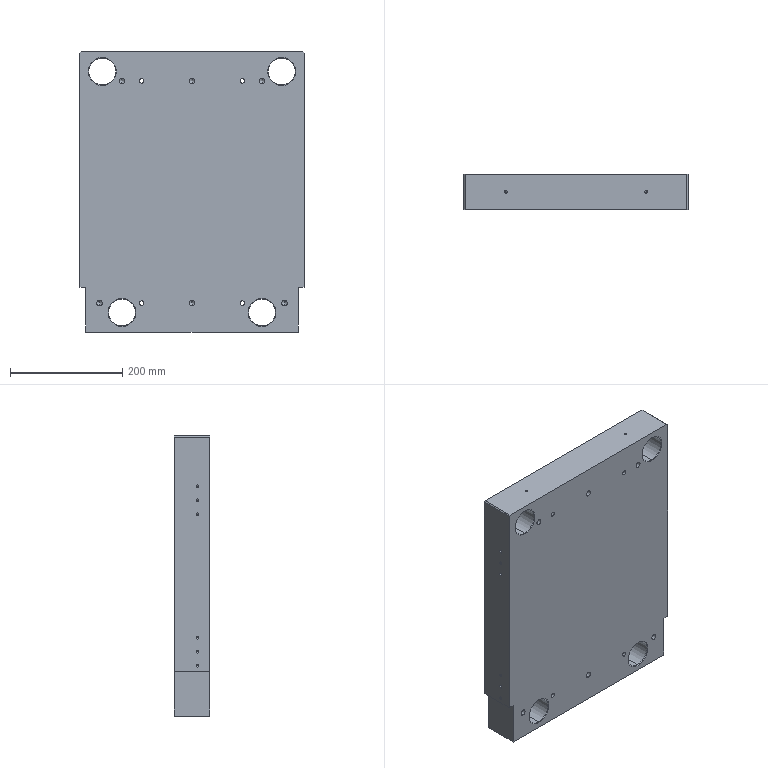Component | SolidWorks | NewDieSet-1_UpperDieSetAssembly-1_KF525R2-MJ-A001-1 | 1 solid | 136 faces | box 400 x 63 x 500 mm | volume 12000457 mm3 | cylinder 64 | cone 60 | plane 12 | commonest cylinder face diameters 5 x32 10.2 x12 8 x8 48 x8 14 x4 | material 55
build123d program:
from build123d import *

# Parameters (mm, degrees)
SKETCH1_W                   = 400
SKETCH1_H                   = 500
BOSS_EXTRUDE1_DEPTH         = 63
SKETCH3_R                   = 24
CUT_EXTRUDE2_DEPTH          = 644.404
CHAMFER1_SIZE               = 1
M6_TAPPED_HOLE1_AT_2_COUNT  = 2
M6_TAPPED_HOLE1_AT_2_PITCH  = 50
M6_TAPPED_HOLE1_AT_3_COUNT  = 2
M6_TAPPED_HOLE1_AT_3_PITCH  = 25
M16_TAPPED_HOLE1_D          = 14
M16_TAPPED_HOLE1_DEPTH      = 30
M16_TAPPED_HOLE1_TIP        = 4.206
M12_TAPPED_HOLE2_AT_2_COUNT = 2
M12_TAPPED_HOLE2_AT_2_PITCH = 165
M12_TAPPED_HOLE2_AT_3_COUNT = 2
M12_TAPPED_HOLE2_AT_3_PITCH = 330
SKETCH45_R                  = 4
CUT_EXTRUDE15_DEPTH         = 644.404
CHAMFER3_SIZE               = 2
SKETCH50_W                  = 10
SKETCH50_H                  = 80
CUT_EXTRUDE17_DEPTH         = 644.404
M6_TAPPED_HOLE3_AT_2_COUNT  = 2
M6_TAPPED_HOLE3_AT_2_PITCH  = 250
M12_TAPPED_HOLE3_D          = 10.2
M12_TAPPED_HOLE3_DEPTH      = 29.25
M12_TAPPED_HOLE3_TIP        = 3.064


with BuildPart() as part:
    # Sketch1 → Boss-Extrude1 (new body)
    with BuildSketch(Plane(origin=(0, 0, 0), x_dir=(1, 0, 0), z_dir=(0, 1, 0))):
        with Locations((200, 250)):
            Rectangle(SKETCH1_W, SKETCH1_H)
    extrude(amount=BOSS_EXTRUDE1_DEPTH)

    # Sketch3 → Cut-Extrude2 (cut, through all)
    with BuildSketch(Plane(origin=(0, 63, 0), x_dir=(1, 0, 0), z_dir=(0, 1, 0))):
        with Locations(Location((75, 465, 0), (0, 0, 270))):
            Circle(SKETCH3_R)
        with Locations(Location((40, 35, 0), (0, 0, 270))):
            Circle(SKETCH3_R)
        with Locations(Location((360, 35, 0), (0, 0, 90))):
            Circle(SKETCH3_R)
        with Locations(Location((325, 465, 0), (0, 0, 90))):
            Circle(SKETCH3_R)
    extrude(amount=-CUT_EXTRUDE2_DEPTH, mode=Mode.SUBTRACT)

    # Chamfer1
    chamfer1_edges = [part.edges().sort_by_distance(p)[0] for p in [
        (75, 0, -489),
        (75, 63, -489),
        (40, 0, -59),
        (40, 63, -59),
        (360, 0, -11),
        (360, 63, -11),
        (325, 0, -441),
        (325, 63, -441),
    ]]
    chamfer(chamfer1_edges, length=CHAMFER1_SIZE)

    # Sketch39 → M6 Tapped Hole1 (revolve, cut)
    with BuildSketch(Plane(origin=(400, 21.5, -140), x_dir=(0, 0, -1), z_dir=(0, 1, 0))):
        Polygon((0, 0), (0, 16.502), (2.5, 15), (2.5, 0), align=None)
    m6_tapped_hole1 = revolve(axis=Axis((406.35, 21.5, -140), (-1, 0, 0)), mode=Mode.SUBTRACT)

    # M6 Tapped Hole1 at 2: M6 Tapped Hole1 ×2
    with Locations(*[(0, 0, i * M6_TAPPED_HOLE1_AT_2_PITCH) for i in range(1, M6_TAPPED_HOLE1_AT_2_COUNT)]):
        add(m6_tapped_hole1, mode=Mode.SUBTRACT)

    # M6 Tapped Hole1 at 3: M6 Tapped Hole1 ×2
    with Locations(*[(0, 0, i * M6_TAPPED_HOLE1_AT_3_PITCH) for i in range(1, M6_TAPPED_HOLE1_AT_3_COUNT)]):
        add(m6_tapped_hole1, mode=Mode.SUBTRACT)

    # Mirror5: M6 Tapped Hole1 across plane
    add(m6_tapped_hole1.mirror(Plane.XY.offset(-250)), mode=Mode.SUBTRACT)

    # Mirror5 copy 1 sketch → Mirror5 copy 1 (revolve, cut)
    with BuildSketch(Plane(origin=(400, 21.5, -410), x_dir=(0, 0, 1), z_dir=(0, 1, 0))):
        Polygon((0, 0), (0, -16.502), (2.5, -15), (2.5, 0), align=None)
    revolve(axis=Axis((406.35, 21.5, -410), (1, 0, 0)), mode=Mode.SUBTRACT)

    # Mirror5 copy 2 sketch → Mirror5 copy 2 (revolve, cut)
    with BuildSketch(Plane(origin=(400, 21.5, -385), x_dir=(0, 0, 1), z_dir=(0, 1, 0))):
        Polygon((0, 0), (0, -16.502), (2.5, -15), (2.5, 0), align=None)
    revolve(axis=Axis((406.35, 21.5, -385), (1, 0, 0)), mode=Mode.SUBTRACT)

    # Mirror6: M6 Tapped Hole1 across plane
    add(m6_tapped_hole1.mirror(Plane.ZY.offset(-200)), mode=Mode.SUBTRACT)

    # Mirror6 copy 1 sketch → Mirror6 copy 1 (revolve, cut)
    with BuildSketch(Plane(origin=(0, 21.5, -90), x_dir=(0, 0, -1), z_dir=(0, 1, 0))):
        Polygon((0, 0), (0, -16.502), (2.5, -15), (2.5, 0), align=None)
    revolve(axis=Axis((-6.35, 21.5, -90), (-1, 0, 0)), mode=Mode.SUBTRACT)

    # Mirror6 copy 2 sketch → Mirror6 copy 2 (revolve, cut)
    with BuildSketch(Plane(origin=(0, 21.5, -115), x_dir=(0, 0, -1), z_dir=(0, 1, 0))):
        Polygon((0, 0), (0, -16.502), (2.5, -15), (2.5, 0), align=None)
    revolve(axis=Axis((-6.35, 21.5, -115), (-1, 0, 0)), mode=Mode.SUBTRACT)

    # Mirror6 copy 3 sketch → Mirror6 copy 3 (revolve, cut)
    with BuildSketch(Plane(origin=(0, 21.5, -360), x_dir=(0, 0, 1), z_dir=(0, 1, 0))):
        Polygon((0, 0), (0, 16.502), (2.5, 15), (2.5, 0), align=None)
    revolve(axis=Axis((-6.35, 21.5, -360), (1, 0, 0)), mode=Mode.SUBTRACT)

    # Mirror6 copy 4 sketch → Mirror6 copy 4 (revolve, cut)
    with BuildSketch(Plane(origin=(0, 21.5, -410), x_dir=(0, 0, 1), z_dir=(0, 1, 0))):
        Polygon((0, 0), (0, 16.502), (2.5, 15), (2.5, 0), align=None)
    revolve(axis=Axis((-6.35, 21.5, -410), (1, 0, 0)), mode=Mode.SUBTRACT)

    # Mirror6 copy 5 sketch → Mirror6 copy 5 (revolve, cut)
    with BuildSketch(Plane(origin=(0, 21.5, -385), x_dir=(0, 0, 1), z_dir=(0, 1, 0))):
        Polygon((0, 0), (0, 16.502), (2.5, 15), (2.5, 0), align=None)
    revolve(axis=Axis((-6.35, 21.5, -385), (1, 0, 0)), mode=Mode.SUBTRACT)

    # M16 Tapped Hole1
    with Locations(Plane(origin=(0, 63, 0), x_dir=(1, 0, 0), z_dir=(0, 1, 0))):
        with Locations((340, 260), (60, 260)):
            Hole(M16_TAPPED_HOLE1_D / 2, depth=M16_TAPPED_HOLE1_DEPTH)
            with Locations((0, 0, -(M16_TAPPED_HOLE1_DEPTH + M16_TAPPED_HOLE1_TIP / 2))):  # 118° drill point
                Cone(0, M16_TAPPED_HOLE1_D / 2, M16_TAPPED_HOLE1_TIP, mode=Mode.SUBTRACT)

    # Sketch43 → M12 Tapped Hole2 (revolve, cut)
    with BuildSketch(Plane(origin=(365, 0, -51.9), x_dir=(0, 0, -1), z_dir=(1, 0, 0))):
        Polygon((0, 0), (0, 32.314), (5.1, 29.25), (5.1, 0), align=None)
    m12_tapped_hole2 = revolve(axis=Axis((365, -6.35, -51.9), (0, 1, 0)), mode=Mode.SUBTRACT)

    # M12 Tapped Hole2 at 2: M12 Tapped Hole2 ×2
    with Locations(*[(-i * M12_TAPPED_HOLE2_AT_2_PITCH, 0, 0) for i in range(1, M12_TAPPED_HOLE2_AT_2_COUNT)]):
        add(m12_tapped_hole2, mode=Mode.SUBTRACT)

    # M12 Tapped Hole2 at 3: M12 Tapped Hole2 ×2
    with Locations(*[(-i * M12_TAPPED_HOLE2_AT_3_PITCH, 0, 0) for i in range(1, M12_TAPPED_HOLE2_AT_3_COUNT)]):
        add(m12_tapped_hole2, mode=Mode.SUBTRACT)

    # Sketch45 → Cut-Extrude15 (cut, through all)
    with BuildSketch(Plane.XZ):
        with Locations(Location((290, -51.9, 0), (0, 0, 270))):
            Circle(SKETCH45_R)
        with Locations(Location((110, -51.9, 0), (0, 0, 270))):
            Circle(SKETCH45_R)
    cut_extrude15 = extrude(amount=-CUT_EXTRUDE15_DEPTH, mode=Mode.SUBTRACT)

    # Mirror7: M12 Tapped Hole2, Cut-Extrude15 across plane
    add(m12_tapped_hole2.mirror(Plane.XY.offset(-250)), mode=Mode.SUBTRACT)
    add(cut_extrude15.mirror(Plane.XY.offset(-250)), mode=Mode.SUBTRACT)

    # Mirror7 copy 1 sketch → Mirror7 copy 1 (revolve, cut)
    with BuildSketch(Plane(origin=(200, 0, -448.1), x_dir=(0, 0, 1), z_dir=(1, 0, 0))):
        Polygon((0, 0), (0, -32.314), (5.1, -29.25), (5.1, 0), align=None)
    revolve(axis=Axis((200, -6.35, -448.1), (0, -1, 0)), mode=Mode.SUBTRACT)

    # Mirror7 copy 2 sketch → Mirror7 copy 2 (revolve, cut)
    with BuildSketch(Plane(origin=(35, 0, -448.1), x_dir=(0, 0, 1), z_dir=(1, 0, 0))):
        Polygon((0, 0), (0, -32.314), (5.1, -29.25), (5.1, 0), align=None)
    revolve(axis=Axis((35, -6.35, -448.1), (0, -1, 0)), mode=Mode.SUBTRACT)

    # Chamfer3
    chamfer3_edges = [part.edges().sort_by_distance(p)[0] for p in [
        (0, 31.5, -500),
        (400, 31.5, -500),
        (400, 31.5, 0),
        (0, 31.5, 0),
    ]]
    chamfer(chamfer3_edges, length=CHAMFER3_SIZE)

    # Sketch50 → Cut-Extrude17 (cut, through all)
    with BuildSketch(Plane(origin=(0, 63, 0), x_dir=(1, 0, 0), z_dir=(0, 1, 0))):
        with Locations((395, 460)):
            Rectangle(SKETCH50_W, SKETCH50_H)
    cut_extrude17 = extrude(amount=-CUT_EXTRUDE17_DEPTH, mode=Mode.SUBTRACT)

    # Mirror9: Cut-Extrude17 across plane
    add(cut_extrude17.mirror(Plane.ZY.offset(-200)), mode=Mode.SUBTRACT)

    # Sketch51 → M6 Tapped Hole3 (revolve, cut)
    with BuildSketch(Plane(origin=(75, 31.5, -500), x_dir=(0, 1, 0), z_dir=(1, 0, 0))):
        Polygon((0, 0), (0, 16.502), (2.5, 15), (2.5, 0), align=None)
    m6_tapped_hole3 = revolve(axis=Axis((75, 31.5, -506.35), (0, 0, 1)), mode=Mode.SUBTRACT)

    # M6 Tapped Hole3 at 2: M6 Tapped Hole3 ×2
    with Locations(*[(i * M6_TAPPED_HOLE3_AT_2_PITCH, 0, 0) for i in range(1, M6_TAPPED_HOLE3_AT_2_COUNT)]):
        add(m6_tapped_hole3, mode=Mode.SUBTRACT)

    # Mirror10: M6 Tapped Hole3 across plane
    add(m6_tapped_hole3.mirror(Plane.XY.offset(-250)), mode=Mode.SUBTRACT)

    # Mirror10 copy 1 sketch → Mirror10 copy 1 (revolve, cut)
    with BuildSketch(Plane(origin=(325, 31.5, 0), x_dir=(0, 1, 0), z_dir=(1, 0, 0))):
        Polygon((0, 0), (0, -16.502), (2.5, -15), (2.5, 0), align=None)
    revolve(axis=Axis((325, 31.5, 6.35), (0, 0, 1)), mode=Mode.SUBTRACT)

    # M12 Tapped Hole3
    with Locations(Plane(origin=(0, 0, 0), x_dir=(-1, 0, 0), z_dir=(0, -1, 0))):
        with Locations((-75, 51.9), (-325, 51.9)):
            Hole(M12_TAPPED_HOLE3_D / 2, depth=M12_TAPPED_HOLE3_DEPTH)
            with Locations((0, 0, -(M12_TAPPED_HOLE3_DEPTH + M12_TAPPED_HOLE3_TIP / 2))):  # 118° drill point
                Cone(0, M12_TAPPED_HOLE3_D / 2, M12_TAPPED_HOLE3_TIP, mode=Mode.SUBTRACT)


solid = part.part

# Placed as in the assembly
solid = solid.moved(Location((-256.746, 95.927, 603), (0, 0, 0)))